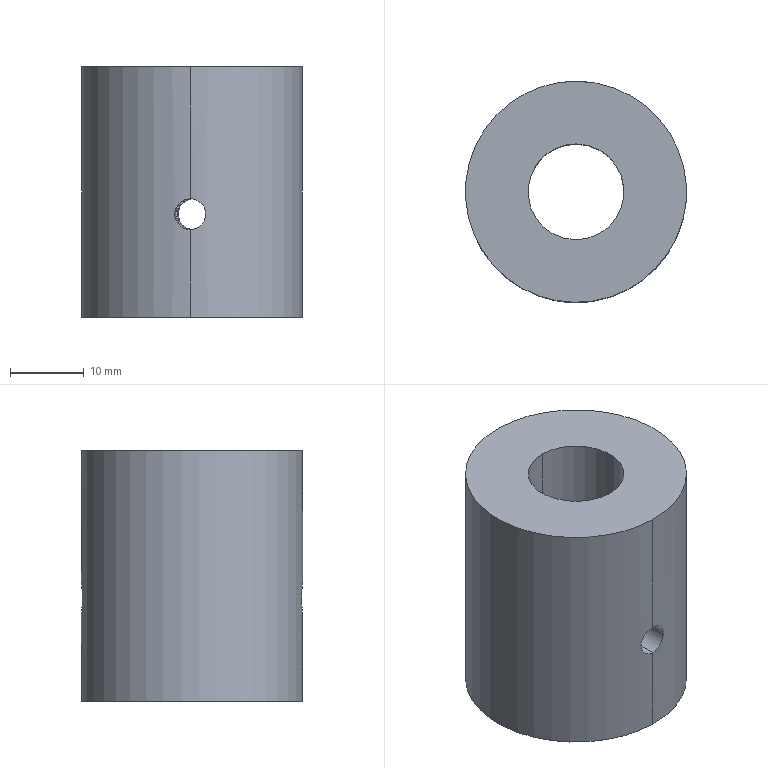Component | SolidWorks | 75-02-15MotorSleeveAxis-1 | 1 solid | 26 faces | box 30 x 30 x 34 mm | volume 18684 mm3 | cylinder 16 | cone 8 | plane 2 | commonest cylinder face diameters 4.2 x12 13 x2 30 x2 | material A3 Steel
build123d program:
from build123d import *

# Parameters (mm, degrees)
SKETCH1_R           = 15
SKETCH1_R_2         = 6.5
BOSS_EXTRUDE1_DEPTH = 17
M5_TAPPED_HOLE1_D   = 4.2
CIRPATTERN1_COUNT   = 4


with BuildPart() as part:
    # Sketch1 → Boss-Extrude1 (new, symmetric)
    with BuildSketch(Plane.XY):
        Circle(SKETCH1_R)
        Circle(SKETCH1_R_2, mode=Mode.SUBTRACT)
    extrude(amount=BOSS_EXTRUDE1_DEPTH, both=True)

    # M5 Tapped Hole1 (through all)
    with Locations(Plane(origin=(15, 0, 3), x_dir=(0, 1, 0), z_dir=(1, 0, 0))):
        with Locations((0, 0)):
            Hole(M5_TAPPED_HOLE1_D / 2)

    # Sketch6 → M5 Tapped Hole2 (revolve, cut)
    with BuildSketch(Plane(origin=(10, 0, 17), x_dir=(0, -1, 0), z_dir=(1, 0, 0))):
        Polygon((0, 0), (0, 11.662), (2.1, 10.4), (2.1, 0), align=None)
    m5_tapped_hole2 = revolve(axis=Axis((10, 0, 23.35), (0, 0, -1)), mode=Mode.SUBTRACT)

    # CirPattern1: M5 Tapped Hole2 ×4 about axis
    cirpattern1_axis = Axis((0, 0, 0), (0, 0, 1))
    for i in range(1, CIRPATTERN1_COUNT):
        add(m5_tapped_hole2.rotate(cirpattern1_axis, i * 360 / CIRPATTERN1_COUNT), mode=Mode.SUBTRACT)


solid = part.part

# Placed as in the assembly
solid = solid.moved(Location((-17.8, 11.867, 93.25), (180, -0.0007069, 90.952)))
STEP:
#1=COLOUR_RGB('',0.7922,0.8196,0.9333);
#2=FILL_AREA_STYLE_COLOUR('',#1);
#3=FILL_AREA_STYLE('',(#2));
#4=SURFACE_STYLE_FILL_AREA(#3);
#5=SURFACE_SIDE_STYLE('',(#4));
#6=SURFACE_STYLE_USAGE(.BOTH.,#5);
#7=PRESENTATION_STYLE_ASSIGNMENT((#6));
#8=CARTESIAN_POINT('',(-0.3085,0.378,3.411));
#9=VERTEX_POINT('',#8);
#10=CARTESIAN_POINT('',(-0.3058,0.5433,3.411));
#11=VERTEX_POINT('',#10);
#12=CARTESIAN_POINT('',(-0.3072,0.4607,3.411));
#13=DIRECTION('',(0.,0.,-1.));
#14=DIRECTION('',(0.0166,0.9999,0.));
#15=AXIS2_PLACEMENT_3D('',#12,#13,#14);
#16=CIRCLE('',#15,0.08268);
#17=EDGE_CURVE('',#9,#11,#16,.T.);
#18=ORIENTED_EDGE('',*,*,#17,.F.);
#19=CARTESIAN_POINT('',(-0.3085,0.378,3.002));
#20=VERTEX_POINT('',#19);
#21=CARTESIAN_POINT('',(-0.3085,0.378,3.002));
#22=DIRECTION('',(0.,0.,-1.));
#23=VECTOR('',#22,39.37);
#24=LINE('',#21,#23);
#25=EDGE_CURVE('',#9,#20,#24,.T.);
#26=ORIENTED_EDGE('',*,*,#25,.T.);
#27=CARTESIAN_POINT('',(-0.3058,0.5433,3.002));
#28=VERTEX_POINT('',#27);
#29=CARTESIAN_POINT('',(-0.3072,0.4607,3.002));
#30=DIRECTION('',(0.,0.,-1.));
#31=DIRECTION('',(0.0166,0.9999,0.));
#32=AXIS2_PLACEMENT_3D('',#29,#30,#31);
#33=CIRCLE('',#32,0.08268);
#34=EDGE_CURVE('',#20,#28,#33,.T.);
#35=ORIENTED_EDGE('',*,*,#34,.T.);
#36=CARTESIAN_POINT('',(-0.3058,0.5433,3.002));
#37=DIRECTION('',(0.,0.,-1.));
#38=VECTOR('',#37,39.37);
#39=LINE('',#36,#38);
#40=EDGE_CURVE('',#11,#28,#39,.T.);
#41=ORIENTED_EDGE('',*,*,#40,.F.);
#42=EDGE_LOOP('',(#18,#26,#35,#41));
#43=FACE_OUTER_BOUND('',#42,.T.);
#44=CARTESIAN_POINT('',(-0.3072,0.4607,3.002));
#45=DIRECTION('',(0.,0.,-1.));
#46=DIRECTION('',(0.0166,0.9999,0.));
#47=AXIS2_PLACEMENT_3D('',#44,#45,#46);
#48=CYLINDRICAL_SURFACE('',#47,0.08268);
#49=ADVANCED_FACE('',(#43),#48,.F.);
#50=CARTESIAN_POINT('',(-0.3072,0.4607,3.461));
#51=VERTEX_POINT('',#50);
#52=CARTESIAN_POINT('',(-0.3058,0.5433,3.411));
#53=DIRECTION('',(0.01423,0.857,-0.515));
#54=VECTOR('',#53,39.37);
#55=LINE('',#52,#54);
#56=EDGE_CURVE('',#51,#11,#55,.T.);
#57=ORIENTED_EDGE('',*,*,#56,.F.);
#58=CARTESIAN_POINT('',(-0.3085,0.378,3.411));
#59=DIRECTION('',(-0.01423,-0.857,-0.515));
#60=VECTOR('',#59,39.37);
#61=LINE('',#58,#60);
#62=EDGE_CURVE('',#51,#9,#61,.T.);
#63=ORIENTED_EDGE('',*,*,#62,.T.);
#64=ORIENTED_EDGE('',*,*,#17,.T.);
#65=EDGE_LOOP('',(#57,#63,#64));
#66=FACE_OUTER_BOUND('',#65,.T.);
#67=CARTESIAN_POINT('',(-0.3072,0.4607,3.411));
#68=DIRECTION('',(0.,0.,-1.));
#69=DIRECTION('',(0.0166,0.9999,0.));
#70=AXIS2_PLACEMENT_3D('',#67,#68,#69);
#71=CONICAL_SURFACE('',#70,0.08268,1.03);
#72=ADVANCED_FACE('',(#66),#71,.F.);
#73=CARTESIAN_POINT('',(-0.7087,-0.009112,3.411));
#74=VERTEX_POINT('',#73);
#75=CARTESIAN_POINT('',(-0.706,0.1562,3.411));
#76=VERTEX_POINT('',#75);
#77=CARTESIAN_POINT('',(-0.7073,0.07355,3.411));
#78=DIRECTION('',(0.,0.,-1.));
#79=DIRECTION('',(0.0166,0.9999,0.));
#80=AXIS2_PLACEMENT_3D('',#77,#78,#79);
#81=CIRCLE('',#80,0.08268);
#82=EDGE_CURVE('',#74,#76,#81,.T.);
#83=ORIENTED_EDGE('',*,*,#82,.F.);
#84=CARTESIAN_POINT('',(-0.7087,-0.009112,3.002));
#85=VERTEX_POINT('',#84);
#86=CARTESIAN_POINT('',(-0.7087,-0.009112,3.002));
#87=DIRECTION('',(0.,0.,-1.));
#88=VECTOR('',#87,39.37);
#89=LINE('',#86,#88);
#90=EDGE_CURVE('',#74,#85,#89,.T.);
#91=ORIENTED_EDGE('',*,*,#90,.T.);
#92=CARTESIAN_POINT('',(-0.706,0.1562,3.002));
#93=VERTEX_POINT('',#92);
#94=CARTESIAN_POINT('',(-0.7073,0.07355,3.002));
#95=DIRECTION('',(0.,0.,-1.));
#96=DIRECTION('',(0.0166,0.9999,0.));
#97=AXIS2_PLACEMENT_3D('',#94,#95,#96);
#98=CIRCLE('',#97,0.08268);
#99=EDGE_CURVE('',#85,#93,#98,.T.);
#100=ORIENTED_EDGE('',*,*,#99,.T.);
#101=CARTESIAN_POINT('',(-0.706,0.1562,3.002));
#102=DIRECTION('',(0.,0.,-1.));
#103=VECTOR('',#102,39.37);
#104=LINE('',#101,#103);
#105=EDGE_CURVE('',#76,#93,#104,.T.);
#106=ORIENTED_EDGE('',*,*,#105,.F.);
#107=EDGE_LOOP('',(#83,#91,#100,#106));
#108=FACE_OUTER_BOUND('',#107,.T.);
#109=CARTESIAN_POINT('',(-0.7073,0.07355,3.002));
#110=DIRECTION('',(0.,0.,-1.));
#111=DIRECTION('',(0.0166,0.9999,0.));
#112=AXIS2_PLACEMENT_3D('',#109,#110,#111);
#113=CYLINDRICAL_SURFACE('',#112,0.08268);
#114=ADVANCED_FACE('',(#108),#113,.F.);
#115=CARTESIAN_POINT('',(-0.7073,0.07355,3.461));
#116=VERTEX_POINT('',#115);
#117=CARTESIAN_POINT('',(-0.706,0.1562,3.411));
#118=DIRECTION('',(0.01423,0.857,-0.515));
#119=VECTOR('',#118,39.37);
#120=LINE('',#117,#119);
#121=EDGE_CURVE('',#116,#76,#120,.T.);
#122=ORIENTED_EDGE('',*,*,#121,.F.);
#123=CARTESIAN_POINT('',(-0.7087,-0.009112,3.411));
#124=DIRECTION('',(-0.01423,-0.857,-0.515));
#125=VECTOR('',#124,39.37);
#126=LINE('',#123,#125);
#127=EDGE_CURVE('',#116,#74,#126,.T.);
#128=ORIENTED_EDGE('',*,*,#127,.T.);
#129=ORIENTED_EDGE('',*,*,#82,.T.);
#130=EDGE_LOOP('',(#122,#128,#129));
#131=FACE_OUTER_BOUND('',#130,.T.);
#132=CARTESIAN_POINT('',(-0.7073,0.07355,3.411));
#133=DIRECTION('',(0.,0.,-1.));
#134=DIRECTION('',(0.0166,0.9999,0.));
#135=AXIS2_PLACEMENT_3D('',#132,#133,#134);
#136=CONICAL_SURFACE('',#135,0.08268,1.03);
#137=ADVANCED_FACE('',(#131),#136,.F.);
#138=CARTESIAN_POINT('',(-1.096,0.3911,3.411));
#139=VERTEX_POINT('',#138);
#140=CARTESIAN_POINT('',(-1.093,0.5564,3.411));
#141=VERTEX_POINT('',#140);
#142=CARTESIAN_POINT('',(-1.094,0.4737,3.411));
#143=DIRECTION('',(0.,0.,-1.));
#144=DIRECTION('',(0.0166,0.9999,0.));
#145=AXIS2_PLACEMENT_3D('',#142,#143,#144);
#146=CIRCLE('',#145,0.08268);
#147=EDGE_CURVE('',#139,#141,#146,.T.);
#148=ORIENTED_EDGE('',*,*,#147,.F.);
#149=CARTESIAN_POINT('',(-1.096,0.3911,3.002));
#150=VERTEX_POINT('',#149);
#151=CARTESIAN_POINT('',(-1.096,0.3911,3.002));
#152=DIRECTION('',(0.,0.,-1.));
#153=VECTOR('',#152,39.37);
#154=LINE('',#151,#153);
#155=EDGE_CURVE('',#139,#150,#154,.T.);
#156=ORIENTED_EDGE('',*,*,#155,.T.);
#157=CARTESIAN_POINT('',(-1.093,0.5564,3.002));
#158=VERTEX_POINT('',#157);
#159=CARTESIAN_POINT('',(-1.094,0.4737,3.002));
#160=DIRECTION('',(0.,0.,-1.));
#161=DIRECTION('',(0.0166,0.9999,0.));
#162=AXIS2_PLACEMENT_3D('',#159,#160,#161);
#163=CIRCLE('',#162,0.08268);
#164=EDGE_CURVE('',#150,#158,#163,.T.);
#165=ORIENTED_EDGE('',*,*,#164,.T.);
#166=CARTESIAN_POINT('',(-1.093,0.5564,3.002));
#167=DIRECTION('',(0.,0.,-1.));
#168=VECTOR('',#167,39.37);
#169=LINE('',#166,#168);
#170=EDGE_CURVE('',#141,#158,#169,.T.);
#171=ORIENTED_EDGE('',*,*,#170,.F.);
#172=EDGE_LOOP('',(#148,#156,#165,#171));
#173=FACE_OUTER_BOUND('',#172,.T.);
#174=CARTESIAN_POINT('',(-1.094,0.4737,3.002));
#175=DIRECTION('',(0.,0.,-1.));
#176=DIRECTION('',(0.0166,0.9999,0.));
#177=AXIS2_PLACEMENT_3D('',#174,#175,#176);
#178=CYLINDRICAL_SURFACE('',#177,0.08268);
#179=ADVANCED_FACE('',(#173),#178,.F.);
#180=CARTESIAN_POINT('',(-1.094,0.4737,3.461));
#181=VERTEX_POINT('',#180);
#182=CARTESIAN_POINT('',(-1.093,0.5564,3.411));
#183=DIRECTION('',(0.01423,0.857,-0.515));
#184=VECTOR('',#183,39.37);
#185=LINE('',#182,#184);
#186=EDGE_CURVE('',#181,#141,#185,.T.);
#187=ORIENTED_EDGE('',*,*,#186,.F.);
#188=CARTESIAN_POINT('',(-1.096,0.3911,3.411));
#189=DIRECTION('',(-0.01423,-0.857,-0.515));
#190=VECTOR('',#189,39.37);
#191=LINE('',#188,#190);
#192=EDGE_CURVE('',#181,#139,#191,.T.);
#193=ORIENTED_EDGE('',*,*,#192,.T.);
#194=ORIENTED_EDGE('',*,*,#147,.T.);
#195=EDGE_LOOP('',(#187,#193,#194));
#196=FACE_OUTER_BOUND('',#195,.T.);
#197=CARTESIAN_POINT('',(-1.094,0.4737,3.411));
#198=DIRECTION('',(0.,0.,-1.));
#199=DIRECTION('',(0.0166,0.9999,0.));
#200=AXIS2_PLACEMENT_3D('',#197,#198,#199);
#201=CONICAL_SURFACE('',#200,0.08268,1.03);
#202=ADVANCED_FACE('',(#196),#201,.F.);
#203=CARTESIAN_POINT('',(-0.6956,0.7782,3.411));
#204=VERTEX_POINT('',#203);
#205=CARTESIAN_POINT('',(-0.6929,0.9435,3.411));
#206=VERTEX_POINT('',#205);
#207=CARTESIAN_POINT('',(-0.6943,0.8608,3.411));
#208=DIRECTION('',(0.,0.,-1.));
#209=DIRECTION('',(0.0166,0.9999,0.));
#210=AXIS2_PLACEMENT_3D('',#207,#208,#209);
#211=CIRCLE('',#210,0.08268);
#212=EDGE_CURVE('',#204,#206,#211,.T.);
#213=ORIENTED_EDGE('',*,*,#212,.F.);
#214=CARTESIAN_POINT('',(-0.6956,0.7782,3.002));
#215=VERTEX_POINT('',#214);
#216=CARTESIAN_POINT('',(-0.6956,0.7782,3.002));
#217=DIRECTION('',(0.,0.,-1.));
#218=VECTOR('',#217,39.37);
#219=LINE('',#216,#218);
#220=EDGE_CURVE('',#204,#215,#219,.T.);
#221=ORIENTED_EDGE('',*,*,#220,.T.);
#222=CARTESIAN_POINT('',(-0.6929,0.9435,3.002));
#223=VERTEX_POINT('',#222);
#224=CARTESIAN_POINT('',(-0.6943,0.8608,3.002));
#225=DIRECTION('',(0.,0.,-1.));
#226=DIRECTION('',(0.0166,0.9999,0.));
#227=AXIS2_PLACEMENT_3D('',#224,#225,#226);
#228=CIRCLE('',#227,0.08268);
#229=EDGE_CURVE('',#215,#223,#228,.T.);
#230=ORIENTED_EDGE('',*,*,#229,.T.);
#231=CARTESIAN_POINT('',(-0.6929,0.9435,3.002));
#232=DIRECTION('',(0.,0.,-1.));
#233=VECTOR('',#232,39.37);
#234=LINE('',#231,#233);
#235=EDGE_CURVE('',#206,#223,#234,.T.);
#236=ORIENTED_EDGE('',*,*,#235,.F.);
#237=EDGE_LOOP('',(#213,#221,#230,#236));
#238=FACE_OUTER_BOUND('',#237,.T.);
#239=CARTESIAN_POINT('',(-0.6943,0.8608,3.002));
#240=DIRECTION('',(0.,0.,-1.));
#241=DIRECTION('',(0.0166,0.9999,0.));
#242=AXIS2_PLACEMENT_3D('',#239,#240,#241);
#243=CYLINDRICAL_SURFACE('',#242,0.08268);
#244=ADVANCED_FACE('',(#238),#243,.F.);
#245=CARTESIAN_POINT('',(-0.6943,0.8608,3.461));
#246=VERTEX_POINT('',#245);
#247=CARTESIAN_POINT('',(-0.6929,0.9435,3.411));
#248=DIRECTION('',(0.01423,0.857,-0.515));
#249=VECTOR('',#248,39.37);
#250=LINE('',#247,#249);
#251=EDGE_CURVE('',#246,#206,#250,.T.);
#252=ORIENTED_EDGE('',*,*,#251,.F.);
#253=CARTESIAN_POINT('',(-0.6956,0.7782,3.411));
#254=DIRECTION('',(-0.01423,-0.857,-0.515));
#255=VECTOR('',#254,39.37);
#256=LINE('',#253,#255);
#257=EDGE_CURVE('',#246,#204,#256,.T.);
#258=ORIENTED_EDGE('',*,*,#257,.T.);
#259=ORIENTED_EDGE('',*,*,#212,.T.);
#260=EDGE_LOOP('',(#252,#258,#259));
#261=FACE_OUTER_BOUND('',#260,.T.);
#262=CARTESIAN_POINT('',(-0.6943,0.8608,3.411));
#263=DIRECTION('',(0.,0.,-1.));
#264=DIRECTION('',(0.0166,0.9999,0.));
#265=AXIS2_PLACEMENT_3D('',#262,#263,#264);
#266=CONICAL_SURFACE('',#265,0.08268,1.03);
#267=ADVANCED_FACE('',(#261),#266,.F.);
#268=CARTESIAN_POINT('',(-0.7106,-0.1233,3.47));
#269=VERTEX_POINT('',#268);
#270=CARTESIAN_POINT('',(-0.7106,-0.1233,3.636));
#271=VERTEX_POINT('',#270);
#272=CARTESIAN_POINT('',(-0.7106,-0.1233,3.47));
#273=CARTESIAN_POINT('',(-0.7214,-0.1231,3.47));
#274=CARTESIAN_POINT('',(-0.7323,-0.1226,3.473));
#275=CARTESIAN_POINT('',(-0.7472,-0.1215,3.479));
#276=CARTESIAN_POINT('',(-0.752,-0.1211,3.481));
#277=CARTESIAN_POINT('',(-0.761,-0.1203,3.487));
#278=CARTESIAN_POINT('',(-0.7652,-0.1198,3.491));
#279=CARTESIAN_POINT('',(-0.7728,-0.119,3.498));
#280=CARTESIAN_POINT('',(-0.7763,-0.1185,3.503));
#281=CARTESIAN_POINT('',(-0.7822,-0.1177,3.512));
#282=CARTESIAN_POINT('',(-0.7848,-0.1174,3.516));
#283=CARTESIAN_POINT('',(-0.7889,-0.1167,3.526));
#284=CARTESIAN_POINT('',(-0.7905,-0.1165,3.532));
#285=CARTESIAN_POINT('',(-0.7926,-0.1162,3.542));
#286=CARTESIAN_POINT('',(-0.7932,-0.1161,3.548));
#287=CARTESIAN_POINT('',(-0.7932,-0.1161,3.559));
#288=CARTESIAN_POINT('',(-0.7926,-0.1162,3.564));
#289=CARTESIAN_POINT('',(-0.7906,-0.1165,3.575));
#290=CARTESIAN_POINT('',(-0.789,-0.1167,3.58));
#291=CARTESIAN_POINT('',(-0.7848,-0.1173,3.59));
#292=CARTESIAN_POINT('',(-0.7823,-0.1177,3.595));
#293=CARTESIAN_POINT('',(-0.7763,-0.1185,3.604));
#294=CARTESIAN_POINT('',(-0.7728,-0.119,3.608));
#295=CARTESIAN_POINT('',(-0.7615,-0.1203,3.619));
#296=CARTESIAN_POINT('',(-0.7523,-0.1212,3.625));
#297=CARTESIAN_POINT('',(-0.7324,-0.1226,3.634));
#298=CARTESIAN_POINT('',(-0.7215,-0.1231,3.636));
#299=CARTESIAN_POINT('',(-0.7106,-0.1233,3.636));
#300=B_SPLINE_CURVE_WITH_KNOTS('',3,(#272,#273,#274,#275,#276,#277,#278,#279,#280,#281,#282,#283,#284,#285,#286,#287,#288,#289,#290,#291,#292,#293,#294,#295,#296,#297,#298,#299),.UNSPECIFIED.,.F.,.F.,(4,2,2,2,2,2,2,2,2,2,2,2,2,4),(0.006574,0.007395,0.007806,0.008217,0.008627,0.009038,0.009449,0.00986,0.01027,0.01068,0.01109,0.0115,0.01232,0.01315),.UNSPECIFIED.);
#301=EDGE_CURVE('',#269,#271,#300,.T.);
#302=ORIENTED_EDGE('',*,*,#301,.F.);
#303=CARTESIAN_POINT('',(-0.705,0.2113,3.47));
#304=VERTEX_POINT('',#303);
#305=CARTESIAN_POINT('',(-0.691,1.058,3.47));
#306=DIRECTION('',(0.0166,0.9999,0.));
#307=VECTOR('',#306,39.37);
#308=LINE('',#305,#307);
#309=EDGE_CURVE('',#269,#304,#308,.T.);
#310=ORIENTED_EDGE('',*,*,#309,.T.);
#311=CARTESIAN_POINT('',(-0.705,0.2113,3.636));
#312=VERTEX_POINT('',#311);
#313=CARTESIAN_POINT('',(-0.705,0.2113,3.47));
#314=CARTESIAN_POINT('',(-0.7105,0.2114,3.47));
#315=CARTESIAN_POINT('',(-0.7159,0.2117,3.471));
#316=CARTESIAN_POINT('',(-0.7266,0.2125,3.473));
#317=CARTESIAN_POINT('',(-0.7318,0.2131,3.475));
#318=CARTESIAN_POINT('',(-0.7418,0.2145,3.479));
#319=CARTESIAN_POINT('',(-0.7465,0.2154,3.481));
#320=CARTESIAN_POINT('',(-0.7554,0.2172,3.487));
#321=CARTESIAN_POINT('',(-0.7596,0.2181,3.491));
#322=CARTESIAN_POINT('',(-0.771,0.221,3.502));
#323=CARTESIAN_POINT('',(-0.7771,0.2229,3.511));
#324=CARTESIAN_POINT('',(-0.7832,0.2249,3.526));
#325=CARTESIAN_POINT('',(-0.7848,0.2255,3.532));
#326=CARTESIAN_POINT('',(-0.787,0.2262,3.542));
#327=CARTESIAN_POINT('',(-0.7875,0.2264,3.548));
#328=CARTESIAN_POINT('',(-0.7875,0.2264,3.559));
#329=CARTESIAN_POINT('',(-0.7869,0.2262,3.564));
#330=CARTESIAN_POINT('',(-0.7848,0.2255,3.575));
#331=CARTESIAN_POINT('',(-0.7833,0.2249,3.58));
#332=CARTESIAN_POINT('',(-0.7791,0.2236,3.59));
#333=CARTESIAN_POINT('',(-0.7765,0.2227,3.595));
#334=CARTESIAN_POINT('',(-0.7706,0.221,3.604));
#335=CARTESIAN_POINT('',(-0.7672,0.22,3.608));
#336=CARTESIAN_POINT('',(-0.7596,0.2181,3.615));
#337=CARTESIAN_POINT('',(-0.7555,0.2172,3.619));
#338=CARTESIAN_POINT('',(-0.7465,0.2154,3.625));
#339=CARTESIAN_POINT('',(-0.7417,0.2145,3.627));
#340=CARTESIAN_POINT('',(-0.7318,0.2131,3.632));
#341=CARTESIAN_POINT('',(-0.7266,0.2125,3.633));
#342=CARTESIAN_POINT('',(-0.7159,0.2117,3.635));
#343=CARTESIAN_POINT('',(-0.7105,0.2114,3.636));
#344=CARTESIAN_POINT('',(-0.705,0.2113,3.636));
#345=B_SPLINE_CURVE_WITH_KNOTS('',3,(#313,#314,#315,#316,#317,#318,#319,#320,#321,#322,#323,#324,#325,#326,#327,#328,#329,#330,#331,#332,#333,#334,#335,#336,#337,#338,#339,#340,#341,#342,#343,#344),.UNSPECIFIED.,.F.,.F.,(4,2,2,2,2,2,2,2,2,2,2,2,2,2,2,4),(0.,0.0004131,0.0008263,0.001239,0.001653,0.002479,0.002892,0.003305,0.003718,0.004131,0.004545,0.004958,0.005371,0.005784,0.006197,0.00661),.UNSPECIFIED.);
#346=EDGE_CURVE('',#304,#312,#345,.T.);
#347=ORIENTED_EDGE('',*,*,#346,.T.);
#348=CARTESIAN_POINT('',(-0.691,1.058,3.636));
#349=DIRECTION('',(0.0166,0.9999,0.));
#350=VECTOR('',#349,39.37);
#351=LINE('',#348,#350);
#352=EDGE_CURVE('',#271,#312,#351,.T.);
#353=ORIENTED_EDGE('',*,*,#352,.F.);
#354=EDGE_LOOP('',(#302,#310,#347,#353));
#355=FACE_OUTER_BOUND('',#354,.T.);
#356=CARTESIAN_POINT('',(-0.691,1.058,3.553));
#357=DIRECTION('',(0.0166,0.9999,0.));
#358=DIRECTION('',(0.,0.,1.));
#359=AXIS2_PLACEMENT_3D('',#356,#357,#358);
#360=CYLINDRICAL_SURFACE('',#359,0.08268);
#361=ADVANCED_FACE('',(#355),#360,.F.);
#362=CARTESIAN_POINT('',(-0.6966,0.7231,3.636));
#363=VERTEX_POINT('',#362);
#364=CARTESIAN_POINT('',(-0.6966,0.7231,3.47));
#365=VERTEX_POINT('',#364);
#366=CARTESIAN_POINT('',(-0.6966,0.7231,3.636));
#367=CARTESIAN_POINT('',(-0.7021,0.7232,3.636));
#368=CARTESIAN_POINT('',(-0.7075,0.7231,3.635));
#369=CARTESIAN_POINT('',(-0.7181,0.7226,3.633));
#370=CARTESIAN_POINT('',(-0.7234,0.7222,3.632));
#371=CARTESIAN_POINT('',(-0.7334,0.7211,3.627));
#372=CARTESIAN_POINT('',(-0.7381,0.7204,3.625));
#373=CARTESIAN_POINT('',(-0.7471,0.7189,3.619));
#374=CARTESIAN_POINT('',(-0.7513,0.7181,3.615));
#375=CARTESIAN_POINT('',(-0.7627,0.7156,3.604));
#376=CARTESIAN_POINT('',(-0.7689,0.7139,3.595));
#377=CARTESIAN_POINT('',(-0.7751,0.7121,3.58));
#378=CARTESIAN_POINT('',(-0.7768,0.7116,3.575));
#379=CARTESIAN_POINT('',(-0.7789,0.7109,3.564));
#380=CARTESIAN_POINT('',(-0.7794,0.7107,3.559));
#381=CARTESIAN_POINT('',(-0.7794,0.7107,3.548));
#382=CARTESIAN_POINT('',(-0.7789,0.7109,3.542));
#383=CARTESIAN_POINT('',(-0.7768,0.7116,3.532));
#384=CARTESIAN_POINT('',(-0.7752,0.7121,3.526));
#385=CARTESIAN_POINT('',(-0.771,0.7133,3.516));
#386=CARTESIAN_POINT('',(-0.7684,0.714,3.512));
#387=CARTESIAN_POINT('',(-0.7624,0.7156,3.503));
#388=CARTESIAN_POINT('',(-0.7589,0.7164,3.498));
#389=CARTESIAN_POINT('',(-0.7513,0.7181,3.491));
#390=CARTESIAN_POINT('',(-0.7471,0.7189,3.487));
#391=CARTESIAN_POINT('',(-0.7382,0.7204,3.481));
#392=CARTESIAN_POINT('',(-0.7333,0.7211,3.479));
#393=CARTESIAN_POINT('',(-0.7233,0.7222,3.475));
#394=CARTESIAN_POINT('',(-0.7182,0.7226,3.473));
#395=CARTESIAN_POINT('',(-0.7075,0.7231,3.471));
#396=CARTESIAN_POINT('',(-0.702,0.7232,3.47));
#397=CARTESIAN_POINT('',(-0.6966,0.7231,3.47));
#398=B_SPLINE_CURVE_WITH_KNOTS('',3,(#366,#367,#368,#369,#370,#371,#372,#373,#374,#375,#376,#377,#378,#379,#380,#381,#382,#383,#384,#385,#386,#387,#388,#389,#390,#391,#392,#393,#394,#395,#396,#397),.UNSPECIFIED.,.F.,.F.,(4,2,2,2,2,2,2,2,2,2,2,2,2,2,2,4),(0.,0.0004131,0.0008263,0.001239,0.001653,0.002479,0.002892,0.003305,0.003718,0.004131,0.004545,0.004958,0.005371,0.005784,0.006197,0.00661),.UNSPECIFIED.);
#399=EDGE_CURVE('',#363,#365,#398,.T.);
#400=ORIENTED_EDGE('',*,*,#399,.T.);
#401=CARTESIAN_POINT('',(-0.691,1.058,3.47));
#402=VERTEX_POINT('',#401);
#403=CARTESIAN_POINT('',(-0.691,1.058,3.47));
#404=DIRECTION('',(0.0166,0.9999,0.));
#405=VECTOR('',#404,39.37);
#406=LINE('',#403,#405);
#407=EDGE_CURVE('',#365,#402,#406,.T.);
#408=ORIENTED_EDGE('',*,*,#407,.T.);
#409=CARTESIAN_POINT('',(-0.691,1.058,3.636));
#410=VERTEX_POINT('',#409);
#411=CARTESIAN_POINT('',(-0.691,1.058,3.636));
#412=CARTESIAN_POINT('',(-0.6965,1.058,3.636));
#413=CARTESIAN_POINT('',(-0.7018,1.058,3.635));
#414=CARTESIAN_POINT('',(-0.7124,1.058,3.633));
#415=CARTESIAN_POINT('',(-0.7177,1.058,3.632));
#416=CARTESIAN_POINT('',(-0.7277,1.057,3.627));
#417=CARTESIAN_POINT('',(-0.7325,1.057,3.625));
#418=CARTESIAN_POINT('',(-0.7414,1.056,3.619));
#419=CARTESIAN_POINT('',(-0.7457,1.056,3.615));
#420=CARTESIAN_POINT('',(-0.7571,1.055,3.604));
#421=CARTESIAN_POINT('',(-0.7633,1.054,3.595));
#422=CARTESIAN_POINT('',(-0.7716,1.054,3.575));
#423=CARTESIAN_POINT('',(-0.7738,1.053,3.564));
#424=CARTESIAN_POINT('',(-0.7738,1.053,3.548));
#425=CARTESIAN_POINT('',(-0.7732,1.053,3.542));
#426=CARTESIAN_POINT('',(-0.7711,1.054,3.532));
#427=CARTESIAN_POINT('',(-0.7695,1.054,3.527));
#428=CARTESIAN_POINT('',(-0.7654,1.054,3.517));
#429=CARTESIAN_POINT('',(-0.7628,1.054,3.512));
#430=CARTESIAN_POINT('',(-0.7568,1.055,3.503));
#431=CARTESIAN_POINT('',(-0.7534,1.055,3.499));
#432=CARTESIAN_POINT('',(-0.7456,1.056,3.491));
#433=CARTESIAN_POINT('',(-0.7415,1.056,3.487));
#434=CARTESIAN_POINT('',(-0.7325,1.057,3.481));
#435=CARTESIAN_POINT('',(-0.7277,1.057,3.479));
#436=CARTESIAN_POINT('',(-0.7177,1.058,3.475));
#437=CARTESIAN_POINT('',(-0.7125,1.058,3.473));
#438=CARTESIAN_POINT('',(-0.7019,1.058,3.471));
#439=CARTESIAN_POINT('',(-0.6964,1.058,3.47));
#440=CARTESIAN_POINT('',(-0.691,1.058,3.47));
#441=B_SPLINE_CURVE_WITH_KNOTS('',3,(#411,#412,#413,#414,#415,#416,#417,#418,#419,#420,#421,#422,#423,#424,#425,#426,#427,#428,#429,#430,#431,#432,#433,#434,#435,#436,#437,#438,#439,#440),.UNSPECIFIED.,.F.,.F.,(4,2,2,2,2,2,2,2,2,2,2,2,2,2,4),(0.,0.0004109,0.0008217,0.001233,0.001643,0.002465,0.003287,0.003698,0.004109,0.004519,0.00493,0.005341,0.005752,0.006163,0.006574),.UNSPECIFIED.);
#442=EDGE_CURVE('',#410,#402,#441,.T.);
#443=ORIENTED_EDGE('',*,*,#442,.F.);
#444=CARTESIAN_POINT('',(-0.691,1.058,3.636));
#445=DIRECTION('',(0.0166,0.9999,0.));
#446=VECTOR('',#445,39.37);
#447=LINE('',#444,#446);
#448=EDGE_CURVE('',#363,#410,#447,.T.);
#449=ORIENTED_EDGE('',*,*,#448,.F.);
#450=EDGE_LOOP('',(#400,#408,#443,#449));
#451=FACE_OUTER_BOUND('',#450,.T.);
#452=CARTESIAN_POINT('',(-0.691,1.058,3.553));
#453=DIRECTION('',(0.0166,0.9999,0.));
#454=DIRECTION('',(0.,0.,1.));
#455=AXIS2_PLACEMENT_3D('',#452,#453,#454);
#456=CYLINDRICAL_SURFACE('',#455,0.08268);
#457=ADVANCED_FACE('',(#451),#456,.F.);
#458=CARTESIAN_POINT('',(-0.705,0.2113,3.002));
#459=VERTEX_POINT('',#458);
#460=CARTESIAN_POINT('',(-0.6966,0.7231,3.002));
#461=VERTEX_POINT('',#460);
#462=CARTESIAN_POINT('',(-0.7008,0.4672,3.002));
#463=DIRECTION('',(0.,0.,-1.));
#464=DIRECTION('',(0.0166,0.9999,0.));
#465=AXIS2_PLACEMENT_3D('',#462,#463,#464);
#466=CIRCLE('',#465,0.2559);
#467=EDGE_CURVE('',#459,#461,#466,.T.);
#468=ORIENTED_EDGE('',*,*,#467,.T.);
#469=CARTESIAN_POINT('',(-0.6966,0.7231,3.002));
#470=DIRECTION('',(-0.,-0.,1.));
#471=VECTOR('',#470,39.37);
#472=LINE('',#469,#471);
#473=EDGE_CURVE('',#461,#365,#472,.T.);
#474=ORIENTED_EDGE('',*,*,#473,.T.);
#475=ORIENTED_EDGE('',*,*,#399,.F.);
#476=CARTESIAN_POINT('',(-0.6966,0.7231,4.341));
#477=VERTEX_POINT('',#476);
#478=CARTESIAN_POINT('',(-0.6966,0.7231,3.002));
#479=DIRECTION('',(-0.,-0.,1.));
#480=VECTOR('',#479,39.37);
#481=LINE('',#478,#480);
#482=EDGE_CURVE('',#363,#477,#481,.T.);
#483=ORIENTED_EDGE('',*,*,#482,.T.);
#484=CARTESIAN_POINT('',(-0.705,0.2113,4.341));
#485=VERTEX_POINT('',#484);
#486=CARTESIAN_POINT('',(-0.7008,0.4672,4.341));
#487=DIRECTION('',(0.,0.,-1.));
#488=DIRECTION('',(0.0166,0.9999,0.));
#489=AXIS2_PLACEMENT_3D('',#486,#487,#488);
#490=CIRCLE('',#489,0.2559);
#491=EDGE_CURVE('',#485,#477,#490,.T.);
#492=ORIENTED_EDGE('',*,*,#491,.F.);
#493=CARTESIAN_POINT('',(-0.705,0.2113,3.002));
#494=DIRECTION('',(-0.,-0.,1.));
#495=VECTOR('',#494,39.37);
#496=LINE('',#493,#495);
#497=EDGE_CURVE('',#312,#485,#496,.T.);
#498=ORIENTED_EDGE('',*,*,#497,.F.);
#499=ORIENTED_EDGE('',*,*,#346,.F.);
#500=CARTESIAN_POINT('',(-0.705,0.2113,3.002));
#501=DIRECTION('',(-0.,-0.,1.));
#502=VECTOR('',#501,39.37);
#503=LINE('',#500,#502);
#504=EDGE_CURVE('',#459,#304,#503,.T.);
#505=ORIENTED_EDGE('',*,*,#504,.F.);
#506=EDGE_LOOP('',(#468,#474,#475,#483,#492,#498,#499,#505));
#507=FACE_OUTER_BOUND('',#506,.T.);
#508=CARTESIAN_POINT('',(-0.7008,0.4672,3.002));
#509=DIRECTION('',(-0.,-0.,1.));
#510=DIRECTION('',(-0.0166,-0.9999,0.));
#511=AXIS2_PLACEMENT_3D('',#508,#509,#510);
#512=CYLINDRICAL_SURFACE('',#511,0.2559);
#513=ADVANCED_FACE('',(#507),#512,.F.);
#514=CARTESIAN_POINT('',(-0.691,1.058,3.002));
#515=VERTEX_POINT('',#514);
#516=CARTESIAN_POINT('',(-0.7106,-0.1233,3.002));
#517=VERTEX_POINT('',#516);
#518=CARTESIAN_POINT('',(-0.7008,0.4672,3.002));
#519=DIRECTION('',(0.,0.,-1.));
#520=DIRECTION('',(0.0166,0.9999,0.));
#521=AXIS2_PLACEMENT_3D('',#518,#519,#520);
#522=CIRCLE('',#521,0.5906);
#523=EDGE_CURVE('',#515,#517,#522,.T.);
#524=ORIENTED_EDGE('',*,*,#523,.F.);
#525=CARTESIAN_POINT('',(-0.691,1.058,3.002));
#526=DIRECTION('',(-0.,-0.,1.));
#527=VECTOR('',#526,39.37);
#528=LINE('',#525,#527);
#529=EDGE_CURVE('',#515,#402,#528,.T.);
#530=ORIENTED_EDGE('',*,*,#529,.T.);
#531=CARTESIAN_POINT('',(-0.691,1.058,3.47));
#532=CARTESIAN_POINT('',(-0.6802,1.057,3.47));
#533=CARTESIAN_POINT('',(-0.6693,1.057,3.473));
#534=CARTESIAN_POINT('',(-0.6544,1.056,3.479));
#535=CARTESIAN_POINT('',(-0.6496,1.056,3.481));
#536=CARTESIAN_POINT('',(-0.6406,1.055,3.487));
#537=CARTESIAN_POINT('',(-0.6364,1.054,3.491));
#538=CARTESIAN_POINT('',(-0.6288,1.053,3.498));
#539=CARTESIAN_POINT('',(-0.6253,1.053,3.503));
#540=CARTESIAN_POINT('',(-0.6194,1.052,3.512));
#541=CARTESIAN_POINT('',(-0.6168,1.052,3.516));
#542=CARTESIAN_POINT('',(-0.6127,1.051,3.526));
#543=CARTESIAN_POINT('',(-0.6111,1.051,3.532));
#544=CARTESIAN_POINT('',(-0.609,1.051,3.542));
#545=CARTESIAN_POINT('',(-0.6084,1.05,3.548));
#546=CARTESIAN_POINT('',(-0.6084,1.05,3.559));
#547=CARTESIAN_POINT('',(-0.609,1.051,3.564));
#548=CARTESIAN_POINT('',(-0.611,1.051,3.575));
#549=CARTESIAN_POINT('',(-0.6126,1.051,3.58));
#550=CARTESIAN_POINT('',(-0.6168,1.052,3.59));
#551=CARTESIAN_POINT('',(-0.6193,1.052,3.595));
#552=CARTESIAN_POINT('',(-0.6253,1.053,3.604));
#553=CARTESIAN_POINT('',(-0.6288,1.053,3.608));
#554=CARTESIAN_POINT('',(-0.6401,1.055,3.619));
#555=CARTESIAN_POINT('',(-0.6493,1.056,3.625));
#556=CARTESIAN_POINT('',(-0.6692,1.057,3.634));
#557=CARTESIAN_POINT('',(-0.6801,1.057,3.636));
#558=CARTESIAN_POINT('',(-0.691,1.058,3.636));
#559=B_SPLINE_CURVE_WITH_KNOTS('',3,(#531,#532,#533,#534,#535,#536,#537,#538,#539,#540,#541,#542,#543,#544,#545,#546,#547,#548,#549,#550,#551,#552,#553,#554,#555,#556,#557,#558),.UNSPECIFIED.,.F.,.F.,(4,2,2,2,2,2,2,2,2,2,2,2,2,4),(0.006574,0.007395,0.007806,0.008217,0.008627,0.009038,0.009449,0.00986,0.01027,0.01068,0.01109,0.0115,0.01232,0.01315),.UNSPECIFIED.);
#560=EDGE_CURVE('',#402,#410,#559,.T.);
#561=ORIENTED_EDGE('',*,*,#560,.T.);
#562=CARTESIAN_POINT('',(-0.691,1.058,4.341));
#563=VERTEX_POINT('',#562);
#564=CARTESIAN_POINT('',(-0.691,1.058,3.002));
#565=DIRECTION('',(-0.,-0.,1.));
#566=VECTOR('',#565,39.37);
#567=LINE('',#564,#566);
#568=EDGE_CURVE('',#410,#563,#567,.T.);
#569=ORIENTED_EDGE('',*,*,#568,.T.);
#570=CARTESIAN_POINT('',(-0.7106,-0.1233,4.341));
#571=VERTEX_POINT('',#570);
#572=CARTESIAN_POINT('',(-0.7008,0.4672,4.341));
#573=DIRECTION('',(0.,0.,-1.));
#574=DIRECTION('',(0.0166,0.9999,0.));
#575=AXIS2_PLACEMENT_3D('',#572,#573,#574);
#576=CIRCLE('',#575,0.5906);
#577=EDGE_CURVE('',#563,#571,#576,.T.);
#578=ORIENTED_EDGE('',*,*,#577,.T.);
#579=CARTESIAN_POINT('',(-0.7106,-0.1233,3.002));
#580=DIRECTION('',(-0.,-0.,1.));
#581=VECTOR('',#580,39.37);
#582=LINE('',#579,#581);
#583=EDGE_CURVE('',#271,#571,#582,.T.);
#584=ORIENTED_EDGE('',*,*,#583,.F.);
#585=CARTESIAN_POINT('',(-0.7106,-0.1233,3.636));
#586=CARTESIAN_POINT('',(-0.7051,-0.1234,3.636));
#587=CARTESIAN_POINT('',(-0.6998,-0.1234,3.635));
#588=CARTESIAN_POINT('',(-0.6892,-0.1233,3.633));
#589=CARTESIAN_POINT('',(-0.6839,-0.1231,3.632));
#590=CARTESIAN_POINT('',(-0.6739,-0.1228,3.627));
#591=CARTESIAN_POINT('',(-0.6691,-0.1225,3.625));
#592=CARTESIAN_POINT('',(-0.6602,-0.122,3.619));
#593=CARTESIAN_POINT('',(-0.6559,-0.1217,3.615));
#594=CARTESIAN_POINT('',(-0.6445,-0.1207,3.604));
#595=CARTESIAN_POINT('',(-0.6383,-0.12,3.595));
#596=CARTESIAN_POINT('',(-0.63,-0.1191,3.575));
#597=CARTESIAN_POINT('',(-0.6278,-0.1188,3.564));
#598=CARTESIAN_POINT('',(-0.6278,-0.1188,3.548));
#599=CARTESIAN_POINT('',(-0.6284,-0.1189,3.542));
#600=CARTESIAN_POINT('',(-0.6305,-0.1192,3.532));
#601=CARTESIAN_POINT('',(-0.6321,-0.1193,3.527));
#602=CARTESIAN_POINT('',(-0.6362,-0.1198,3.517));
#603=CARTESIAN_POINT('',(-0.6388,-0.1201,3.512));
#604=CARTESIAN_POINT('',(-0.6448,-0.1207,3.503));
#605=CARTESIAN_POINT('',(-0.6482,-0.121,3.499));
#606=CARTESIAN_POINT('',(-0.656,-0.1217,3.491));
#607=CARTESIAN_POINT('',(-0.6601,-0.122,3.487));
#608=CARTESIAN_POINT('',(-0.6691,-0.1225,3.481));
#609=CARTESIAN_POINT('',(-0.6739,-0.1228,3.479));
#610=CARTESIAN_POINT('',(-0.6839,-0.1231,3.475));
#611=CARTESIAN_POINT('',(-0.6891,-0.1233,3.473));
#612=CARTESIAN_POINT('',(-0.6997,-0.1234,3.471));
#613=CARTESIAN_POINT('',(-0.7052,-0.1234,3.47));
#614=CARTESIAN_POINT('',(-0.7106,-0.1233,3.47));
#615=B_SPLINE_CURVE_WITH_KNOTS('',3,(#585,#586,#587,#588,#589,#590,#591,#592,#593,#594,#595,#596,#597,#598,#599,#600,#601,#602,#603,#604,#605,#606,#607,#608,#609,#610,#611,#612,#613,#614),.UNSPECIFIED.,.F.,.F.,(4,2,2,2,2,2,2,2,2,2,2,2,2,2,4),(0.,0.0004109,0.0008217,0.001233,0.001643,0.002465,0.003287,0.003698,0.004109,0.004519,0.00493,0.005341,0.005752,0.006163,0.006574),.UNSPECIFIED.);
#616=EDGE_CURVE('',#271,#269,#615,.T.);
#617=ORIENTED_EDGE('',*,*,#616,.T.);
#618=CARTESIAN_POINT('',(-0.7106,-0.1233,3.002));
#619=DIRECTION('',(-0.,-0.,1.));
#620=VECTOR('',#619,39.37);
#621=LINE('',#618,#620);
#622=EDGE_CURVE('',#517,#269,#621,.T.);
#623=ORIENTED_EDGE('',*,*,#622,.F.);
#624=EDGE_LOOP('',(#524,#530,#561,#569,#578,#584,#617,#623));
#625=FACE_OUTER_BOUND('',#624,.T.);
#626=CARTESIAN_POINT('',(-0.7008,0.4672,3.002));
#627=DIRECTION('',(-0.,-0.,1.));
#628=DIRECTION('',(-0.0166,-0.9999,0.));
#629=AXIS2_PLACEMENT_3D('',#626,#627,#628);
#630=CYLINDRICAL_SURFACE('',#629,0.5906);
#631=ADVANCED_FACE('',(#625),#630,.T.);
#632=CARTESIAN_POINT('',(-0.3072,0.4607,3.002));
#633=DIRECTION('',(0.,0.,-1.));
#634=DIRECTION('',(0.0166,0.9999,0.));
#635=AXIS2_PLACEMENT_3D('',#632,#633,#634);
#636=CIRCLE('',#635,0.08268);
#637=EDGE_CURVE('',#28,#20,#636,.T.);
#638=ORIENTED_EDGE('',*,*,#637,.F.);
#639=ORIENTED_EDGE('',*,*,#34,.F.);
#640=EDGE_LOOP('',(#638,#639));
#641=FACE_BOUND('',#640,.T.);
#642=CARTESIAN_POINT('',(-0.7073,0.07355,3.002));
#643=DIRECTION('',(0.,0.,-1.));
#644=DIRECTION('',(0.0166,0.9999,0.));
#645=AXIS2_PLACEMENT_3D('',#642,#643,#644);
#646=CIRCLE('',#645,0.08268);
#647=EDGE_CURVE('',#93,#85,#646,.T.);
#648=ORIENTED_EDGE('',*,*,#647,.F.);
#649=ORIENTED_EDGE('',*,*,#99,.F.);
#650=EDGE_LOOP('',(#648,#649));
#651=FACE_BOUND('',#650,.T.);
#652=CARTESIAN_POINT('',(-1.094,0.4737,3.002));
#653=DIRECTION('',(0.,0.,-1.));
#654=DIRECTION('',(0.0166,0.9999,0.));
#655=AXIS2_PLACEMENT_3D('',#652,#653,#654);
#656=CIRCLE('',#655,0.08268);
#657=EDGE_CURVE('',#158,#150,#656,.T.);
#658=ORIENTED_EDGE('',*,*,#657,.F.);
#659=ORIENTED_EDGE('',*,*,#164,.F.);
#660=EDGE_LOOP('',(#658,#659));
#661=FACE_BOUND('',#660,.T.);
#662=CARTESIAN_POINT('',(-0.6943,0.8608,3.002));
#663=DIRECTION('',(0.,0.,-1.));
#664=DIRECTION('',(0.0166,0.9999,0.));
#665=AXIS2_PLACEMENT_3D('',#662,#663,#664);
#666=CIRCLE('',#665,0.08268);
#667=EDGE_CURVE('',#223,#215,#666,.T.);
#668=ORIENTED_EDGE('',*,*,#667,.F.);
#669=ORIENTED_EDGE('',*,*,#229,.F.);
#670=EDGE_LOOP('',(#668,#669));
#671=FACE_BOUND('',#670,.T.);
#672=CARTESIAN_POINT('',(-0.7008,0.4672,3.002));
#673=DIRECTION('',(0.,0.,-1.));
#674=DIRECTION('',(0.0166,0.9999,0.));
#675=AXIS2_PLACEMENT_3D('',#672,#673,#674);
#676=CIRCLE('',#675,0.5906);
#677=EDGE_CURVE('',#517,#515,#676,.T.);
#678=ORIENTED_EDGE('',*,*,#677,.T.);
#679=ORIENTED_EDGE('',*,*,#523,.T.);
#680=EDGE_LOOP('',(#678,#679));
#681=FACE_OUTER_BOUND('',#680,.T.);
#682=ORIENTED_EDGE('',*,*,#467,.F.);
#683=CARTESIAN_POINT('',(-0.7008,0.4672,3.002));
#684=DIRECTION('',(0.,0.,-1.));
#685=DIRECTION('',(0.0166,0.9999,0.));
#686=AXIS2_PLACEMENT_3D('',#683,#684,#685);
#687=CIRCLE('',#686,0.2559);
#688=EDGE_CURVE('',#461,#459,#687,.T.);
#689=ORIENTED_EDGE('',*,*,#688,.F.);
#690=EDGE_LOOP('',(#682,#689));
#691=FACE_BOUND('',#690,.T.);
#692=CARTESIAN_POINT('',(-0.7008,0.4672,3.002));
#693=DIRECTION('',(0.,0.,-1.));
#694=DIRECTION('',(0.0166,0.9999,0.));
#695=AXIS2_PLACEMENT_3D('',#692,#693,#694);
#696=PLANE('',#695);
#697=ADVANCED_FACE('',(#641,#651,#661,#671,#681,#691),#696,.T.);
#698=CARTESIAN_POINT('',(-0.7008,0.4672,4.341));
#699=DIRECTION('',(0.,0.,-1.));
#700=DIRECTION('',(0.0166,0.9999,0.));
#701=AXIS2_PLACEMENT_3D('',#698,#699,#700);
#702=CIRCLE('',#701,0.5906);
#703=EDGE_CURVE('',#571,#563,#702,.T.);
#704=ORIENTED_EDGE('',*,*,#703,.F.);
#705=ORIENTED_EDGE('',*,*,#577,.F.);
#706=EDGE_LOOP('',(#704,#705));
#707=FACE_OUTER_BOUND('',#706,.T.);
#708=ORIENTED_EDGE('',*,*,#491,.T.);
#709=CARTESIAN_POINT('',(-0.7008,0.4672,4.341));
#710=DIRECTION('',(0.,0.,-1.));
#711=DIRECTION('',(0.0166,0.9999,0.));
#712=AXIS2_PLACEMENT_3D('',#709,#710,#711);
#713=CIRCLE('',#712,0.2559);
#714=EDGE_CURVE('',#477,#485,#713,.T.);
#715=ORIENTED_EDGE('',*,*,#714,.T.);
#716=EDGE_LOOP('',(#708,#715));
#717=FACE_BOUND('',#716,.T.);
#718=CARTESIAN_POINT('',(-0.7008,0.4672,4.341));
#719=DIRECTION('',(0.,0.,-1.));
#720=DIRECTION('',(0.0166,0.9999,0.));
#721=AXIS2_PLACEMENT_3D('',#718,#719,#720);
#722=PLANE('',#721);
#723=ADVANCED_FACE('',(#707,#717),#722,.F.);
#724=ORIENTED_EDGE('',*,*,#529,.F.);
#725=ORIENTED_EDGE('',*,*,#677,.F.);
#726=ORIENTED_EDGE('',*,*,#622,.T.);
#727=ORIENTED_EDGE('',*,*,#301,.T.);
#728=ORIENTED_EDGE('',*,*,#583,.T.);
#729=ORIENTED_EDGE('',*,*,#703,.T.);
#730=ORIENTED_EDGE('',*,*,#568,.F.);
#731=ORIENTED_EDGE('',*,*,#442,.T.);
#732=EDGE_LOOP('',(#724,#725,#726,#727,#728,#729,#730,#731));
#733=FACE_OUTER_BOUND('',#732,.T.);
#734=CARTESIAN_POINT('',(-0.7008,0.4672,3.002));
#735=DIRECTION('',(-0.,-0.,1.));
#736=DIRECTION('',(-0.0166,-0.9999,0.));
#737=AXIS2_PLACEMENT_3D('',#734,#735,#736);
#738=CYLINDRICAL_SURFACE('',#737,0.5906);
#739=ADVANCED_FACE('',(#733),#738,.T.);
#740=ORIENTED_EDGE('',*,*,#473,.F.);
#741=ORIENTED_EDGE('',*,*,#688,.T.);
#742=ORIENTED_EDGE('',*,*,#504,.T.);
#743=CARTESIAN_POINT('',(-0.705,0.2113,3.636));
#744=CARTESIAN_POINT('',(-0.6942,0.2112,3.636));
#745=CARTESIAN_POINT('',(-0.6833,0.2117,3.634));
#746=CARTESIAN_POINT('',(-0.6683,0.2133,3.627));
#747=CARTESIAN_POINT('',(-0.6634,0.214,3.625));
#748=CARTESIAN_POINT('',(-0.6545,0.2155,3.619));
#749=CARTESIAN_POINT('',(-0.6503,0.2163,3.615));
#750=CARTESIAN_POINT('',(-0.6388,0.2188,3.604));
#751=CARTESIAN_POINT('',(-0.6327,0.2205,3.595));
#752=CARTESIAN_POINT('',(-0.6264,0.2223,3.58));
#753=CARTESIAN_POINT('',(-0.6248,0.2228,3.575));
#754=CARTESIAN_POINT('',(-0.6227,0.2235,3.564));
#755=CARTESIAN_POINT('',(-0.6222,0.2237,3.559));
#756=CARTESIAN_POINT('',(-0.6222,0.2237,3.548));
#757=CARTESIAN_POINT('',(-0.6227,0.2235,3.542));
#758=CARTESIAN_POINT('',(-0.6248,0.2228,3.532));
#759=CARTESIAN_POINT('',(-0.6265,0.2223,3.526));
#760=CARTESIAN_POINT('',(-0.6327,0.2205,3.511));
#761=CARTESIAN_POINT('',(-0.6389,0.2188,3.502));
#762=CARTESIAN_POINT('',(-0.6503,0.2163,3.491));
#763=CARTESIAN_POINT('',(-0.6545,0.2155,3.487));
#764=CARTESIAN_POINT('',(-0.6635,0.214,3.481));
#765=CARTESIAN_POINT('',(-0.6682,0.2133,3.479));
#766=CARTESIAN_POINT('',(-0.6782,0.2122,3.475));
#767=CARTESIAN_POINT('',(-0.6835,0.2118,3.473));
#768=CARTESIAN_POINT('',(-0.6941,0.2113,3.471));
#769=CARTESIAN_POINT('',(-0.6995,0.2112,3.47));
#770=CARTESIAN_POINT('',(-0.705,0.2113,3.47));
#771=B_SPLINE_CURVE_WITH_KNOTS('',3,(#743,#744,#745,#746,#747,#748,#749,#750,#751,#752,#753,#754,#755,#756,#757,#758,#759,#760,#761,#762,#763,#764,#765,#766,#767,#768,#769,#770),.UNSPECIFIED.,.F.,.F.,(4,2,2,2,2,2,2,2,2,2,2,2,2,4),(0.00661,0.007436,0.007849,0.008262,0.009088,0.009501,0.009914,0.01033,0.01074,0.01157,0.01198,0.01239,0.01281,0.01322),.UNSPECIFIED.);
#772=EDGE_CURVE('',#312,#304,#771,.T.);
#773=ORIENTED_EDGE('',*,*,#772,.F.);
#774=ORIENTED_EDGE('',*,*,#497,.T.);
#775=ORIENTED_EDGE('',*,*,#714,.F.);
#776=ORIENTED_EDGE('',*,*,#482,.F.);
#777=CARTESIAN_POINT('',(-0.6966,0.7231,3.47));
#778=CARTESIAN_POINT('',(-0.6857,0.7229,3.47));
#779=CARTESIAN_POINT('',(-0.6748,0.722,3.473));
#780=CARTESIAN_POINT('',(-0.6599,0.7199,3.479));
#781=CARTESIAN_POINT('',(-0.655,0.719,3.481));
#782=CARTESIAN_POINT('',(-0.6461,0.7172,3.487));
#783=CARTESIAN_POINT('',(-0.642,0.7163,3.491));
#784=CARTESIAN_POINT('',(-0.6306,0.7134,3.502));
#785=CARTESIAN_POINT('',(-0.6246,0.7115,3.511));
#786=CARTESIAN_POINT('',(-0.6183,0.7095,3.526));
#787=CARTESIAN_POINT('',(-0.6168,0.7089,3.532));
#788=CARTESIAN_POINT('',(-0.6147,0.7082,3.542));
#789=CARTESIAN_POINT('',(-0.6141,0.708,3.548));
#790=CARTESIAN_POINT('',(-0.6141,0.708,3.559));
#791=CARTESIAN_POINT('',(-0.6146,0.7082,3.564));
#792=CARTESIAN_POINT('',(-0.6168,0.7089,3.575));
#793=CARTESIAN_POINT('',(-0.6184,0.7095,3.58));
#794=CARTESIAN_POINT('',(-0.6245,0.7115,3.595));
#795=CARTESIAN_POINT('',(-0.6307,0.7134,3.604));
#796=CARTESIAN_POINT('',(-0.642,0.7163,3.615));
#797=CARTESIAN_POINT('',(-0.6462,0.7172,3.619));
#798=CARTESIAN_POINT('',(-0.6551,0.719,3.625));
#799=CARTESIAN_POINT('',(-0.6598,0.7199,3.627));
#800=CARTESIAN_POINT('',(-0.6698,0.7213,3.632));
#801=CARTESIAN_POINT('',(-0.675,0.7219,3.633));
#802=CARTESIAN_POINT('',(-0.6856,0.7227,3.635));
#803=CARTESIAN_POINT('',(-0.6911,0.723,3.636));
#804=CARTESIAN_POINT('',(-0.6966,0.7231,3.636));
#805=B_SPLINE_CURVE_WITH_KNOTS('',3,(#777,#778,#779,#780,#781,#782,#783,#784,#785,#786,#787,#788,#789,#790,#791,#792,#793,#794,#795,#796,#797,#798,#799,#800,#801,#802,#803,#804),.UNSPECIFIED.,.F.,.F.,(4,2,2,2,2,2,2,2,2,2,2,2,2,4),(0.00661,0.007436,0.007849,0.008262,0.009088,0.009501,0.009914,0.01033,0.01074,0.01157,0.01198,0.01239,0.01281,0.01322),.UNSPECIFIED.);
#806=EDGE_CURVE('',#365,#363,#805,.T.);
#807=ORIENTED_EDGE('',*,*,#806,.F.);
#808=EDGE_LOOP('',(#740,#741,#742,#773,#774,#775,#776,#807));
#809=FACE_OUTER_BOUND('',#808,.T.);
#810=CARTESIAN_POINT('',(-0.7008,0.4672,3.002));
#811=DIRECTION('',(-0.,-0.,1.));
#812=DIRECTION('',(-0.0166,-0.9999,0.));
#813=AXIS2_PLACEMENT_3D('',#810,#811,#812);
#814=CYLINDRICAL_SURFACE('',#813,0.2559);
#815=ADVANCED_FACE('',(#809),#814,.F.);
#816=ORIENTED_EDGE('',*,*,#407,.F.);
#817=ORIENTED_EDGE('',*,*,#806,.T.);
#818=ORIENTED_EDGE('',*,*,#448,.T.);
#819=ORIENTED_EDGE('',*,*,#560,.F.);
#820=EDGE_LOOP('',(#816,#817,#818,#819));
#821=FACE_OUTER_BOUND('',#820,.T.);
#822=CARTESIAN_POINT('',(-0.691,1.058,3.553));
#823=DIRECTION('',(0.0166,0.9999,0.));
#824=DIRECTION('',(0.,0.,1.));
#825=AXIS2_PLACEMENT_3D('',#822,#823,#824);
#826=CYLINDRICAL_SURFACE('',#825,0.08268);
#827=ADVANCED_FACE('',(#821),#826,.F.);
#828=ORIENTED_EDGE('',*,*,#309,.F.);
#829=ORIENTED_EDGE('',*,*,#616,.F.);
#830=ORIENTED_EDGE('',*,*,#352,.T.);
#831=ORIENTED_EDGE('',*,*,#772,.T.);
#832=EDGE_LOOP('',(#828,#829,#830,#831));
#833=FACE_OUTER_BOUND('',#832,.T.);
#834=CARTESIAN_POINT('',(-0.691,1.058,3.553));
#835=DIRECTION('',(0.0166,0.9999,0.));
#836=DIRECTION('',(0.,0.,1.));
#837=AXIS2_PLACEMENT_3D('',#834,#835,#836);
#838=CYLINDRICAL_SURFACE('',#837,0.08268);
#839=ADVANCED_FACE('',(#833),#838,.F.);
#840=ORIENTED_EDGE('',*,*,#257,.F.);
#841=ORIENTED_EDGE('',*,*,#251,.T.);
#842=CARTESIAN_POINT('',(-0.6943,0.8608,3.411));
#843=DIRECTION('',(0.,0.,-1.));
#844=DIRECTION('',(0.0166,0.9999,0.));
#845=AXIS2_PLACEMENT_3D('',#842,#843,#844);
#846=CIRCLE('',#845,0.08268);
#847=EDGE_CURVE('',#206,#204,#846,.T.);
#848=ORIENTED_EDGE('',*,*,#847,.T.);
#849=EDGE_LOOP('',(#840,#841,#848));
#850=FACE_OUTER_BOUND('',#849,.T.);
#851=CARTESIAN_POINT('',(-0.6943,0.8608,3.411));
#852=DIRECTION('',(0.,0.,-1.));
#853=DIRECTION('',(0.0166,0.9999,0.));
#854=AXIS2_PLACEMENT_3D('',#851,#852,#853);
#855=CONICAL_SURFACE('',#854,0.08268,1.03);
#856=ADVANCED_FACE('',(#850),#855,.F.);
#857=ORIENTED_EDGE('',*,*,#220,.F.);
#858=ORIENTED_EDGE('',*,*,#847,.F.);
#859=ORIENTED_EDGE('',*,*,#235,.T.);
#860=ORIENTED_EDGE('',*,*,#667,.T.);
#861=EDGE_LOOP('',(#857,#858,#859,#860));
#862=FACE_OUTER_BOUND('',#861,.T.);
#863=CARTESIAN_POINT('',(-0.6943,0.8608,3.002));
#864=DIRECTION('',(0.,0.,-1.));
#865=DIRECTION('',(0.0166,0.9999,0.));
#866=AXIS2_PLACEMENT_3D('',#863,#864,#865);
#867=CYLINDRICAL_SURFACE('',#866,0.08268);
#868=ADVANCED_FACE('',(#862),#867,.F.);
#869=ORIENTED_EDGE('',*,*,#192,.F.);
#870=ORIENTED_EDGE('',*,*,#186,.T.);
#871=CARTESIAN_POINT('',(-1.094,0.4737,3.411));
#872=DIRECTION('',(0.,0.,-1.));
#873=DIRECTION('',(0.0166,0.9999,0.));
#874=AXIS2_PLACEMENT_3D('',#871,#872,#873);
#875=CIRCLE('',#874,0.08268);
#876=EDGE_CURVE('',#141,#139,#875,.T.);
#877=ORIENTED_EDGE('',*,*,#876,.T.);
#878=EDGE_LOOP('',(#869,#870,#877));
#879=FACE_OUTER_BOUND('',#878,.T.);
#880=CARTESIAN_POINT('',(-1.094,0.4737,3.411));
#881=DIRECTION('',(0.,0.,-1.));
#882=DIRECTION('',(0.0166,0.9999,0.));
#883=AXIS2_PLACEMENT_3D('',#880,#881,#882);
#884=CONICAL_SURFACE('',#883,0.08268,1.03);
#885=ADVANCED_FACE('',(#879),#884,.F.);
#886=ORIENTED_EDGE('',*,*,#155,.F.);
#887=ORIENTED_EDGE('',*,*,#876,.F.);
#888=ORIENTED_EDGE('',*,*,#170,.T.);
#889=ORIENTED_EDGE('',*,*,#657,.T.);
#890=EDGE_LOOP('',(#886,#887,#888,#889));
#891=FACE_OUTER_BOUND('',#890,.T.);
#892=CARTESIAN_POINT('',(-1.094,0.4737,3.002));
#893=DIRECTION('',(0.,0.,-1.));
#894=DIRECTION('',(0.0166,0.9999,0.));
#895=AXIS2_PLACEMENT_3D('',#892,#893,#894);
#896=CYLINDRICAL_SURFACE('',#895,0.08268);
#897=ADVANCED_FACE('',(#891),#896,.F.);
#898=ORIENTED_EDGE('',*,*,#127,.F.);
#899=ORIENTED_EDGE('',*,*,#121,.T.);
#900=CARTESIAN_POINT('',(-0.7073,0.07355,3.411));
#901=DIRECTION('',(0.,0.,-1.));
#902=DIRECTION('',(0.0166,0.9999,0.));
#903=AXIS2_PLACEMENT_3D('',#900,#901,#902);
#904=CIRCLE('',#903,0.08268);
#905=EDGE_CURVE('',#76,#74,#904,.T.);
#906=ORIENTED_EDGE('',*,*,#905,.T.);
#907=EDGE_LOOP('',(#898,#899,#906));
#908=FACE_OUTER_BOUND('',#907,.T.);
#909=CARTESIAN_POINT('',(-0.7073,0.07355,3.411));
#910=DIRECTION('',(0.,0.,-1.));
#911=DIRECTION('',(0.0166,0.9999,0.));
#912=AXIS2_PLACEMENT_3D('',#909,#910,#911);
#913=CONICAL_SURFACE('',#912,0.08268,1.03);
#914=ADVANCED_FACE('',(#908),#913,.F.);
#915=ORIENTED_EDGE('',*,*,#90,.F.);
#916=ORIENTED_EDGE('',*,*,#905,.F.);
#917=ORIENTED_EDGE('',*,*,#105,.T.);
#918=ORIENTED_EDGE('',*,*,#647,.T.);
#919=EDGE_LOOP('',(#915,#916,#917,#918));
#920=FACE_OUTER_BOUND('',#919,.T.);
#921=CARTESIAN_POINT('',(-0.7073,0.07355,3.002));
#922=DIRECTION('',(0.,0.,-1.));
#923=DIRECTION('',(0.0166,0.9999,0.));
#924=AXIS2_PLACEMENT_3D('',#921,#922,#923);
#925=CYLINDRICAL_SURFACE('',#924,0.08268);
#926=ADVANCED_FACE('',(#920),#925,.F.);
#927=ORIENTED_EDGE('',*,*,#62,.F.);
#928=ORIENTED_EDGE('',*,*,#56,.T.);
#929=CARTESIAN_POINT('',(-0.3072,0.4607,3.411));
#930=DIRECTION('',(0.,0.,-1.));
#931=DIRECTION('',(0.0166,0.9999,0.));
#932=AXIS2_PLACEMENT_3D('',#929,#930,#931);
#933=CIRCLE('',#932,0.08268);
#934=EDGE_CURVE('',#11,#9,#933,.T.);
#935=ORIENTED_EDGE('',*,*,#934,.T.);
#936=EDGE_LOOP('',(#927,#928,#935));
#937=FACE_OUTER_BOUND('',#936,.T.);
#938=CARTESIAN_POINT('',(-0.3072,0.4607,3.411));
#939=DIRECTION('',(0.,0.,-1.));
#940=DIRECTION('',(0.0166,0.9999,0.));
#941=AXIS2_PLACEMENT_3D('',#938,#939,#940);
#942=CONICAL_SURFACE('',#941,0.08268,1.03);
#943=ADVANCED_FACE('',(#937),#942,.F.);
#944=ORIENTED_EDGE('',*,*,#25,.F.);
#945=ORIENTED_EDGE('',*,*,#934,.F.);
#946=ORIENTED_EDGE('',*,*,#40,.T.);
#947=ORIENTED_EDGE('',*,*,#637,.T.);
#948=EDGE_LOOP('',(#944,#945,#946,#947));
#949=FACE_OUTER_BOUND('',#948,.T.);
#950=CARTESIAN_POINT('',(-0.3072,0.4607,3.002));
#951=DIRECTION('',(0.,0.,-1.));
#952=DIRECTION('',(0.0166,0.9999,0.));
#953=AXIS2_PLACEMENT_3D('',#950,#951,#952);
#954=CYLINDRICAL_SURFACE('',#953,0.08268);
#955=ADVANCED_FACE('',(#949),#954,.F.);
#956=CLOSED_SHELL('',(#49,#72,#114,#137,#179,#202,#244,#267,#361,#457,#513,#631,#697,#723,#739,#815,#827,#839,#856,#868,#885,#897,#914,#926,#943,#955));
#957=MANIFOLD_SOLID_BREP('',#956);
#958=STYLED_ITEM('',(#7),#957);
#959=(LENGTH_UNIT()NAMED_UNIT(*)SI_UNIT($,.METRE.));
#960=LENGTH_MEASURE_WITH_UNIT(LENGTH_MEASURE(0.0254),#959);
#961=DIMENSIONAL_EXPONENTS(1.,0.,0.,0.,0.,0.,0.);
#962=(CONVERSION_BASED_UNIT('',#960)LENGTH_UNIT()NAMED_UNIT(#961));
#963=UNCERTAINTY_MEASURE_WITH_UNIT(LENGTH_MEASURE(0.00001),#962,'','');
#964=(NAMED_UNIT(*)PLANE_ANGLE_UNIT()SI_UNIT($,.RADIAN.));
#965=(NAMED_UNIT(*)SI_UNIT($,.STERADIAN.)SOLID_ANGLE_UNIT());
#966=(GEOMETRIC_REPRESENTATION_CONTEXT(3)GLOBAL_UNCERTAINTY_ASSIGNED_CONTEXT((#963))GLOBAL_UNIT_ASSIGNED_CONTEXT((#962,#964,#965))REPRESENTATION_CONTEXT('',''));
#967=MECHANICAL_DESIGN_GEOMETRIC_PRESENTATION_REPRESENTATION('',(#958),#966);
#968=PRESENTATION_LAYER_ASSIGNMENT('','',(#958));
#969=CARTESIAN_POINT('',(0.,0.,0.));
#970=DIRECTION('',(0.,0.,1.));
#971=DIRECTION('',(1.,0.,0.));
#972=AXIS2_PLACEMENT_3D('',#969,#970,#971);
#973=(LENGTH_UNIT()NAMED_UNIT(*)SI_UNIT($,.METRE.));
#974=LENGTH_MEASURE_WITH_UNIT(LENGTH_MEASURE(0.0254),#973);
#975=DIMENSIONAL_EXPONENTS(1.,0.,0.,0.,0.,0.,0.);
#976=(CONVERSION_BASED_UNIT('',#974)LENGTH_UNIT()NAMED_UNIT(#975));
#977=UNCERTAINTY_MEASURE_WITH_UNIT(LENGTH_MEASURE(0.00001),#976,'','');
#978=(NAMED_UNIT(*)PLANE_ANGLE_UNIT()SI_UNIT($,.RADIAN.));
#979=(NAMED_UNIT(*)SI_UNIT($,.STERADIAN.)SOLID_ANGLE_UNIT());
#980=(GEOMETRIC_REPRESENTATION_CONTEXT(3)GLOBAL_UNCERTAINTY_ASSIGNED_CONTEXT((#977))GLOBAL_UNIT_ASSIGNED_CONTEXT((#976,#978,#979))REPRESENTATION_CONTEXT('',''));
#981=ADVANCED_BREP_SHAPE_REPRESENTATION('',(#957,#972),#980);